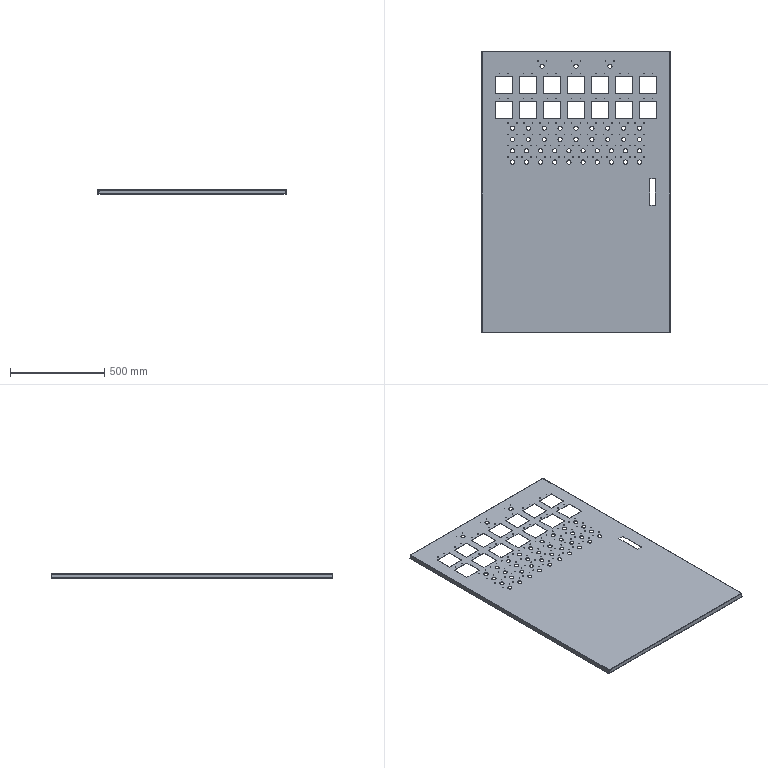Component | SolidWorks | AirFurnaceElectricalCabinet-DoorPanelAssembly-1_AirFurnaceElectricalCabinet-DoorPanel-1 | 1 solid | 440 faces | volume 2277420 mm3 | cylinder 322 | plane 110 | spline 8 | commonest cylinder face diameters 3.4 x220 22.5 x82 1.5 x8 4.5 x8 6.5 x4